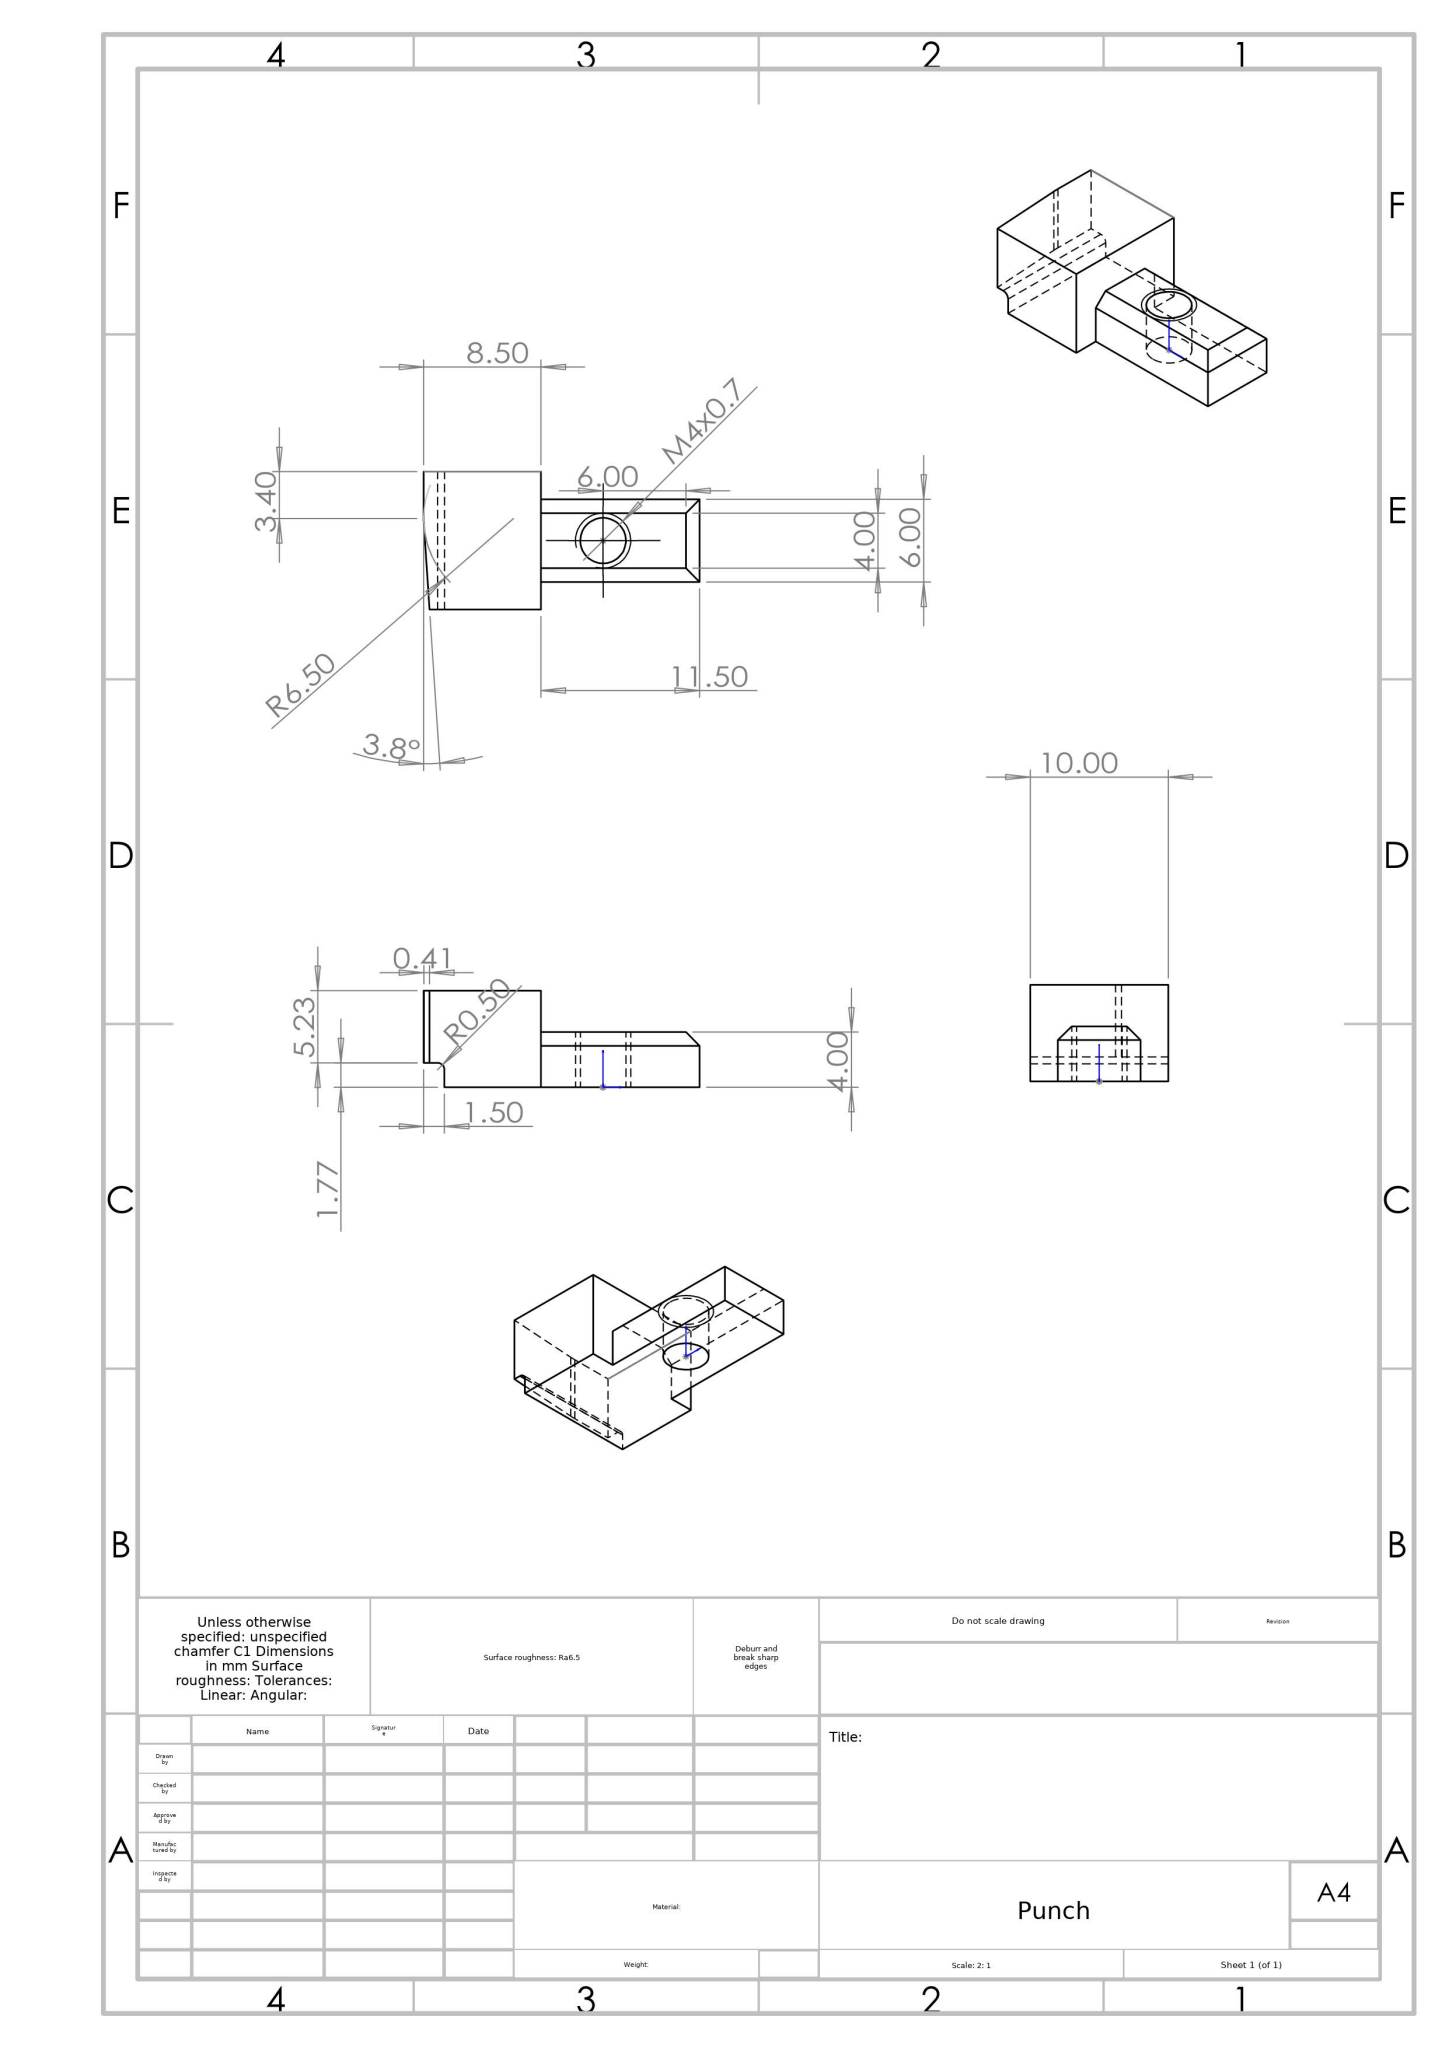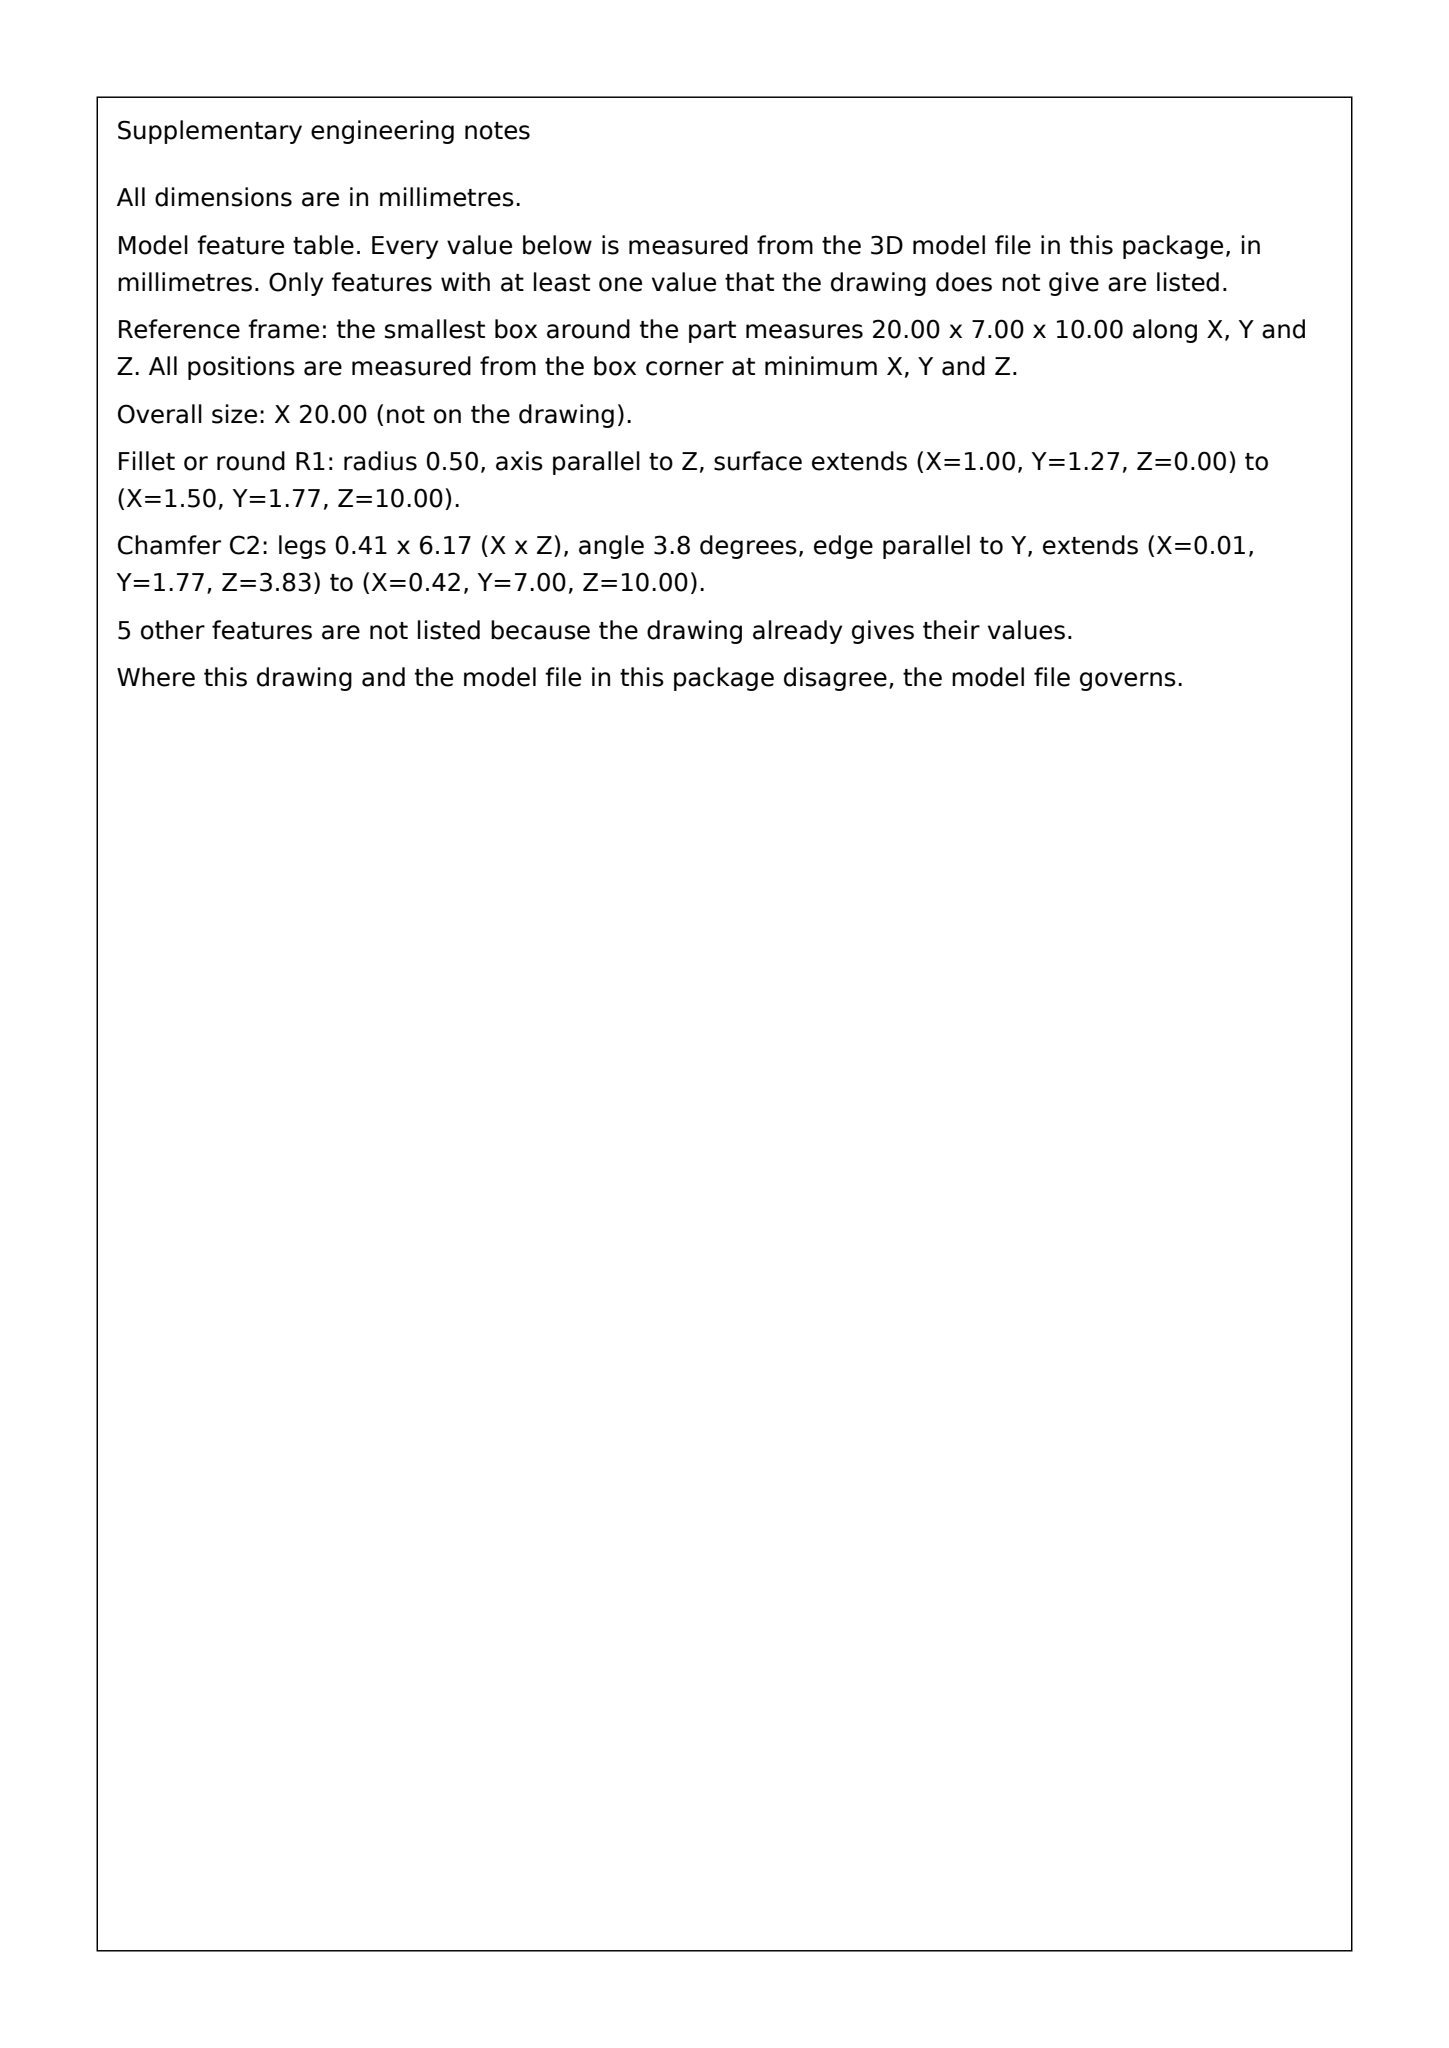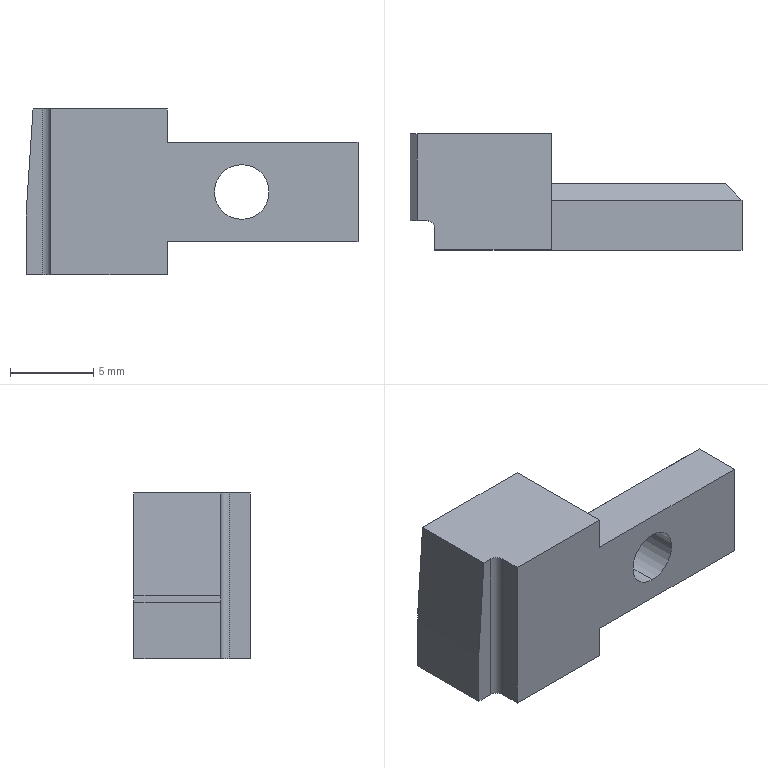Part | SolidWorks | mm | 1 solid | 20 faces | box 20 x 7 x 10 mm | volume 790 mm3 | plane 16 | cylinder 4 | commonest cylinder face diameters 3.3 x2 13 x1 1 x1
STEP:
#1=CARTESIAN_POINT('',(0.,0.,-1.65));
#2=VERTEX_POINT('',#1);
#3=CARTESIAN_POINT('',(0.,0.,1.65));
#4=VERTEX_POINT('',#3);
#5=CARTESIAN_POINT('',(0.,0.,0.));
#6=DIRECTION('',(0.,1.,0.));
#7=DIRECTION('',(0.,0.,1.));
#8=AXIS2_PLACEMENT_3D('',#5,#6,#7);
#9=CIRCLE('',#8,1.65);
#10=EDGE_CURVE('',#2,#4,#9,.T.);
#11=ORIENTED_EDGE('',*,*,#10,.F.);
#12=CARTESIAN_POINT('',(0.,4.,-1.65));
#13=VERTEX_POINT('',#12);
#14=CARTESIAN_POINT('',(0.,4.,-1.65));
#15=DIRECTION('',(0.,1.,0.));
#16=VECTOR('',#15,1000.);
#17=LINE('',#14,#16);
#18=EDGE_CURVE('',#2,#13,#17,.T.);
#19=ORIENTED_EDGE('',*,*,#18,.T.);
#20=CARTESIAN_POINT('',(0.,4.,1.65));
#21=VERTEX_POINT('',#20);
#22=CARTESIAN_POINT('',(0.,4.,0.));
#23=DIRECTION('',(0.,1.,0.));
#24=DIRECTION('',(0.,0.,1.));
#25=AXIS2_PLACEMENT_3D('',#22,#23,#24);
#26=CIRCLE('',#25,1.65);
#27=EDGE_CURVE('',#13,#21,#26,.T.);
#28=ORIENTED_EDGE('',*,*,#27,.T.);
#29=CARTESIAN_POINT('',(0.,4.,1.65));
#30=DIRECTION('',(0.,1.,0.));
#31=VECTOR('',#30,1000.);
#32=LINE('',#29,#31);
#33=EDGE_CURVE('',#4,#21,#32,.T.);
#34=ORIENTED_EDGE('',*,*,#33,.F.);
#35=EDGE_LOOP('',(#11,#19,#28,#34));
#36=FACE_OUTER_BOUND('',#35,.T.);
#37=CARTESIAN_POINT('',(0.,4.,0.));
#38=DIRECTION('',(0.,1.,0.));
#39=DIRECTION('',(0.,0.,1.));
#40=AXIS2_PLACEMENT_3D('',#37,#38,#39);
#41=CYLINDRICAL_SURFACE('',#40,1.65);
#42=ADVANCED_FACE('',(#36),#41,.F.);
#43=CARTESIAN_POINT('',(-13.,7.,-1.6));
#44=VERTEX_POINT('',#43);
#45=CARTESIAN_POINT('',(-12.986,7.,-1.169));
#46=VERTEX_POINT('',#45);
#47=CARTESIAN_POINT('',(-6.5,7.,-1.6));
#48=DIRECTION('',(0.,1.,0.));
#49=DIRECTION('',(0.,0.,1.));
#50=AXIS2_PLACEMENT_3D('',#47,#48,#49);
#51=CIRCLE('',#50,6.5);
#52=EDGE_CURVE('',#44,#46,#51,.T.);
#53=ORIENTED_EDGE('',*,*,#52,.T.);
#54=CARTESIAN_POINT('',(-12.576,7.,5.));
#55=VERTEX_POINT('',#54);
#56=CARTESIAN_POINT('',(-12.852,7.,0.839));
#57=DIRECTION('',(0.06627,0.,0.9978));
#58=VECTOR('',#57,1000.);
#59=LINE('',#56,#58);
#60=EDGE_CURVE('',#46,#55,#59,.T.);
#61=ORIENTED_EDGE('',*,*,#60,.T.);
#62=CARTESIAN_POINT('',(-4.5,7.,5.));
#63=VERTEX_POINT('',#62);
#64=CARTESIAN_POINT('',(-12.78,7.,5.));
#65=DIRECTION('',(1.,0.,0.));
#66=VECTOR('',#65,1000.);
#67=LINE('',#64,#66);
#68=EDGE_CURVE('',#55,#63,#67,.T.);
#69=ORIENTED_EDGE('',*,*,#68,.T.);
#70=CARTESIAN_POINT('',(-4.5,7.,-5.));
#71=VERTEX_POINT('',#70);
#72=CARTESIAN_POINT('',(-4.5,7.,-5.));
#73=DIRECTION('',(0.,0.,-1.));
#74=VECTOR('',#73,1000.);
#75=LINE('',#72,#74);
#76=EDGE_CURVE('',#63,#71,#75,.T.);
#77=ORIENTED_EDGE('',*,*,#76,.T.);
#78=CARTESIAN_POINT('',(-13.,7.,-5.));
#79=VERTEX_POINT('',#78);
#80=CARTESIAN_POINT('',(-12.78,7.,-5.));
#81=DIRECTION('',(1.,0.,0.));
#82=VECTOR('',#81,1000.);
#83=LINE('',#80,#82);
#84=EDGE_CURVE('',#79,#71,#83,.T.);
#85=ORIENTED_EDGE('',*,*,#84,.F.);
#86=CARTESIAN_POINT('',(-13.,7.,-5.));
#87=DIRECTION('',(0.,0.,-1.));
#88=VECTOR('',#87,1000.);
#89=LINE('',#86,#88);
#90=EDGE_CURVE('',#44,#79,#89,.T.);
#91=ORIENTED_EDGE('',*,*,#90,.F.);
#92=EDGE_LOOP('',(#53,#61,#69,#77,#85,#91));
#93=FACE_OUTER_BOUND('',#92,.T.);
#94=CARTESIAN_POINT('',(-12.78,7.,-5.));
#95=DIRECTION('',(0.,-1.,0.));
#96=DIRECTION('',(0.,0.,-1.));
#97=AXIS2_PLACEMENT_3D('',#94,#95,#96);
#98=PLANE('',#97);
#99=ADVANCED_FACE('',(#93),#98,.F.);
#100=CARTESIAN_POINT('',(-12.576,1.77,5.));
#101=VERTEX_POINT('',#100);
#102=CARTESIAN_POINT('',(-12.,1.77,5.));
#103=VERTEX_POINT('',#102);
#104=CARTESIAN_POINT('',(-11.5,1.77,5.));
#105=DIRECTION('',(1.,0.,0.));
#106=VECTOR('',#105,1000.);
#107=LINE('',#104,#106);
#108=EDGE_CURVE('',#101,#103,#107,.T.);
#109=ORIENTED_EDGE('',*,*,#108,.T.);
#110=CARTESIAN_POINT('',(-11.5,1.27,5.));
#111=VERTEX_POINT('',#110);
#112=CARTESIAN_POINT('',(-12.,1.27,5.));
#113=DIRECTION('',(0.,0.,-1.));
#114=DIRECTION('',(-1.,0.,0.));
#115=AXIS2_PLACEMENT_3D('',#112,#113,#114);
#116=CIRCLE('',#115,0.5);
#117=EDGE_CURVE('',#103,#111,#116,.T.);
#118=ORIENTED_EDGE('',*,*,#117,.T.);
#119=CARTESIAN_POINT('',(-11.5,-0.,5.));
#120=VERTEX_POINT('',#119);
#121=CARTESIAN_POINT('',(-11.5,-0.,5.));
#122=DIRECTION('',(0.,-1.,0.));
#123=VECTOR('',#122,1000.);
#124=LINE('',#121,#123);
#125=EDGE_CURVE('',#111,#120,#124,.T.);
#126=ORIENTED_EDGE('',*,*,#125,.T.);
#127=CARTESIAN_POINT('',(-4.5,-0.,5.));
#128=VERTEX_POINT('',#127);
#129=CARTESIAN_POINT('',(-12.78,-0.,5.));
#130=DIRECTION('',(1.,0.,0.));
#131=VECTOR('',#130,1000.);
#132=LINE('',#129,#131);
#133=EDGE_CURVE('',#120,#128,#132,.T.);
#134=ORIENTED_EDGE('',*,*,#133,.T.);
#135=CARTESIAN_POINT('',(-4.5,-0.,5.));
#136=DIRECTION('',(0.,1.,0.));
#137=VECTOR('',#136,1000.);
#138=LINE('',#135,#137);
#139=EDGE_CURVE('',#128,#63,#138,.T.);
#140=ORIENTED_EDGE('',*,*,#139,.T.);
#141=ORIENTED_EDGE('',*,*,#68,.F.);
#142=CARTESIAN_POINT('',(-12.576,-3.,5.));
#143=DIRECTION('',(0.,1.,0.));
#144=VECTOR('',#143,1000.);
#145=LINE('',#142,#144);
#146=EDGE_CURVE('',#101,#55,#145,.T.);
#147=ORIENTED_EDGE('',*,*,#146,.F.);
#148=EDGE_LOOP('',(#109,#118,#126,#134,#140,#141,#147));
#149=FACE_OUTER_BOUND('',#148,.T.);
#150=CARTESIAN_POINT('',(-12.78,-0.,5.));
#151=DIRECTION('',(0.,0.,-1.));
#152=DIRECTION('',(0.,-1.,0.));
#153=AXIS2_PLACEMENT_3D('',#150,#151,#152);
#154=PLANE('',#153);
#155=ADVANCED_FACE('',(#149),#154,.F.);
#156=CARTESIAN_POINT('',(0.,0.,0.));
#157=DIRECTION('',(0.,1.,0.));
#158=DIRECTION('',(0.,0.,1.));
#159=AXIS2_PLACEMENT_3D('',#156,#157,#158);
#160=CIRCLE('',#159,1.65);
#161=EDGE_CURVE('',#4,#2,#160,.T.);
#162=ORIENTED_EDGE('',*,*,#161,.T.);
#163=ORIENTED_EDGE('',*,*,#10,.T.);
#164=EDGE_LOOP('',(#162,#163));
#165=FACE_BOUND('',#164,.T.);
#166=CARTESIAN_POINT('',(-11.5,-0.,-5.));
#167=VERTEX_POINT('',#166);
#168=CARTESIAN_POINT('',(-11.5,-0.,5.));
#169=DIRECTION('',(0.,0.,-1.));
#170=VECTOR('',#169,1000.);
#171=LINE('',#168,#170);
#172=EDGE_CURVE('',#120,#167,#171,.T.);
#173=ORIENTED_EDGE('',*,*,#172,.T.);
#174=CARTESIAN_POINT('',(-4.5,-0.,-5.));
#175=VERTEX_POINT('',#174);
#176=CARTESIAN_POINT('',(-12.78,-0.,-5.));
#177=DIRECTION('',(1.,0.,0.));
#178=VECTOR('',#177,1000.);
#179=LINE('',#176,#178);
#180=EDGE_CURVE('',#167,#175,#179,.T.);
#181=ORIENTED_EDGE('',*,*,#180,.T.);
#182=CARTESIAN_POINT('',(-4.5,0.,-3.));
#183=VERTEX_POINT('',#182);
#184=CARTESIAN_POINT('',(-4.5,-0.,5.));
#185=DIRECTION('',(0.,0.,1.));
#186=VECTOR('',#185,1000.);
#187=LINE('',#184,#186);
#188=EDGE_CURVE('',#175,#183,#187,.T.);
#189=ORIENTED_EDGE('',*,*,#188,.T.);
#190=CARTESIAN_POINT('',(7.,0.,-3.));
#191=VERTEX_POINT('',#190);
#192=CARTESIAN_POINT('',(0.,0.,-3.));
#193=DIRECTION('',(-1.,0.,-0.));
#194=VECTOR('',#193,1000.);
#195=LINE('',#192,#194);
#196=EDGE_CURVE('',#191,#183,#195,.T.);
#197=ORIENTED_EDGE('',*,*,#196,.F.);
#198=CARTESIAN_POINT('',(7.,0.,3.));
#199=VERTEX_POINT('',#198);
#200=CARTESIAN_POINT('',(7.,0.,-3.));
#201=DIRECTION('',(-0.,0.,-1.));
#202=VECTOR('',#201,1000.);
#203=LINE('',#200,#202);
#204=EDGE_CURVE('',#199,#191,#203,.T.);
#205=ORIENTED_EDGE('',*,*,#204,.F.);
#206=CARTESIAN_POINT('',(-4.5,0.,3.));
#207=VERTEX_POINT('',#206);
#208=CARTESIAN_POINT('',(0.,0.,3.));
#209=DIRECTION('',(1.,0.,-0.));
#210=VECTOR('',#209,1000.);
#211=LINE('',#208,#210);
#212=EDGE_CURVE('',#207,#199,#211,.T.);
#213=ORIENTED_EDGE('',*,*,#212,.F.);
#214=CARTESIAN_POINT('',(-4.5,-0.,5.));
#215=DIRECTION('',(0.,0.,1.));
#216=VECTOR('',#215,1000.);
#217=LINE('',#214,#216);
#218=EDGE_CURVE('',#207,#128,#217,.T.);
#219=ORIENTED_EDGE('',*,*,#218,.T.);
#220=ORIENTED_EDGE('',*,*,#133,.F.);
#221=EDGE_LOOP('',(#173,#181,#189,#197,#205,#213,#219,#220));
#222=FACE_OUTER_BOUND('',#221,.T.);
#223=CARTESIAN_POINT('',(0.,0.,0.));
#224=DIRECTION('',(0.,-1.,0.));
#225=DIRECTION('',(0.,0.,-1.));
#226=AXIS2_PLACEMENT_3D('',#223,#224,#225);
#227=PLANE('',#226);
#228=ADVANCED_FACE('',(#165,#222),#227,.T.);
#229=CARTESIAN_POINT('',(-4.5,4.,-2.));
#230=VERTEX_POINT('',#229);
#231=CARTESIAN_POINT('',(-4.5,3.,-3.));
#232=VERTEX_POINT('',#231);
#233=CARTESIAN_POINT('',(-4.5,4.,-2.));
#234=DIRECTION('',(0.,-0.7071,-0.7071));
#235=VECTOR('',#234,1000.);
#236=LINE('',#233,#235);
#237=EDGE_CURVE('',#230,#232,#236,.T.);
#238=ORIENTED_EDGE('',*,*,#237,.T.);
#239=CARTESIAN_POINT('',(-4.5,4.,-3.));
#240=DIRECTION('',(0.,-1.,0.));
#241=VECTOR('',#240,1000.);
#242=LINE('',#239,#241);
#243=EDGE_CURVE('',#232,#183,#242,.T.);
#244=ORIENTED_EDGE('',*,*,#243,.T.);
#245=ORIENTED_EDGE('',*,*,#188,.F.);
#246=CARTESIAN_POINT('',(-4.5,-0.,-5.));
#247=DIRECTION('',(0.,-1.,0.));
#248=VECTOR('',#247,1000.);
#249=LINE('',#246,#248);
#250=EDGE_CURVE('',#71,#175,#249,.T.);
#251=ORIENTED_EDGE('',*,*,#250,.F.);
#252=ORIENTED_EDGE('',*,*,#76,.F.);
#253=ORIENTED_EDGE('',*,*,#139,.F.);
#254=ORIENTED_EDGE('',*,*,#218,.F.);
#255=CARTESIAN_POINT('',(-4.5,3.,3.));
#256=VERTEX_POINT('',#255);
#257=CARTESIAN_POINT('',(-4.5,4.,3.));
#258=DIRECTION('',(0.,-1.,0.));
#259=VECTOR('',#258,1000.);
#260=LINE('',#257,#259);
#261=EDGE_CURVE('',#256,#207,#260,.T.);
#262=ORIENTED_EDGE('',*,*,#261,.F.);
#263=CARTESIAN_POINT('',(-4.5,4.,2.));
#264=VERTEX_POINT('',#263);
#265=CARTESIAN_POINT('',(-4.5,4.,2.));
#266=DIRECTION('',(0.,0.7071,-0.7071));
#267=VECTOR('',#266,1000.);
#268=LINE('',#265,#267);
#269=EDGE_CURVE('',#256,#264,#268,.T.);
#270=ORIENTED_EDGE('',*,*,#269,.T.);
#271=CARTESIAN_POINT('',(-4.5,4.,3.));
#272=DIRECTION('',(0.,0.,1.));
#273=VECTOR('',#272,1000.);
#274=LINE('',#271,#273);
#275=EDGE_CURVE('',#230,#264,#274,.T.);
#276=ORIENTED_EDGE('',*,*,#275,.F.);
#277=EDGE_LOOP('',(#238,#244,#245,#251,#252,#253,#254,#262,#270,#276));
#278=FACE_OUTER_BOUND('',#277,.T.);
#279=CARTESIAN_POINT('',(-4.5,0.,0.));
#280=DIRECTION('',(1.,0.,0.));
#281=DIRECTION('',(0.,1.,0.));
#282=AXIS2_PLACEMENT_3D('',#279,#280,#281);
#283=PLANE('',#282);
#284=ADVANCED_FACE('',(#278),#283,.T.);
#285=CARTESIAN_POINT('',(-13.,1.77,-5.));
#286=VERTEX_POINT('',#285);
#287=CARTESIAN_POINT('',(-13.,-0.,-5.));
#288=DIRECTION('',(0.,-1.,0.));
#289=VECTOR('',#288,1000.);
#290=LINE('',#287,#289);
#291=EDGE_CURVE('',#79,#286,#290,.T.);
#292=ORIENTED_EDGE('',*,*,#291,.T.);
#293=CARTESIAN_POINT('',(-13.,1.77,-1.6));
#294=VERTEX_POINT('',#293);
#295=CARTESIAN_POINT('',(-13.,1.77,5.));
#296=DIRECTION('',(0.,0.,-1.));
#297=VECTOR('',#296,1000.);
#298=LINE('',#295,#297);
#299=EDGE_CURVE('',#294,#286,#298,.T.);
#300=ORIENTED_EDGE('',*,*,#299,.F.);
#301=CARTESIAN_POINT('',(-13.,-3.,-1.6));
#302=DIRECTION('',(0.,1.,0.));
#303=VECTOR('',#302,1000.);
#304=LINE('',#301,#303);
#305=EDGE_CURVE('',#294,#44,#304,.T.);
#306=ORIENTED_EDGE('',*,*,#305,.T.);
#307=ORIENTED_EDGE('',*,*,#90,.T.);
#308=EDGE_LOOP('',(#292,#300,#306,#307));
#309=FACE_OUTER_BOUND('',#308,.T.);
#310=CARTESIAN_POINT('',(-13.,0.,0.));
#311=DIRECTION('',(1.,0.,0.));
#312=DIRECTION('',(0.,1.,0.));
#313=AXIS2_PLACEMENT_3D('',#310,#311,#312);
#314=PLANE('',#313);
#315=ADVANCED_FACE('',(#309),#314,.F.);
#316=ORIENTED_EDGE('',*,*,#180,.F.);
#317=CARTESIAN_POINT('',(-11.5,1.27,-5.));
#318=VERTEX_POINT('',#317);
#319=CARTESIAN_POINT('',(-11.5,-0.,-5.));
#320=DIRECTION('',(0.,-1.,0.));
#321=VECTOR('',#320,1000.);
#322=LINE('',#319,#321);
#323=EDGE_CURVE('',#318,#167,#322,.T.);
#324=ORIENTED_EDGE('',*,*,#323,.F.);
#325=CARTESIAN_POINT('',(-12.,1.77,-5.));
#326=VERTEX_POINT('',#325);
#327=CARTESIAN_POINT('',(-12.,1.27,-5.));
#328=DIRECTION('',(0.,0.,1.));
#329=DIRECTION('',(1.,0.,0.));
#330=AXIS2_PLACEMENT_3D('',#327,#328,#329);
#331=CIRCLE('',#330,0.5);
#332=EDGE_CURVE('',#318,#326,#331,.T.);
#333=ORIENTED_EDGE('',*,*,#332,.T.);
#334=CARTESIAN_POINT('',(-11.5,1.77,-5.));
#335=DIRECTION('',(1.,0.,0.));
#336=VECTOR('',#335,1000.);
#337=LINE('',#334,#336);
#338=EDGE_CURVE('',#286,#326,#337,.T.);
#339=ORIENTED_EDGE('',*,*,#338,.F.);
#340=ORIENTED_EDGE('',*,*,#291,.F.);
#341=ORIENTED_EDGE('',*,*,#84,.T.);
#342=ORIENTED_EDGE('',*,*,#250,.T.);
#343=EDGE_LOOP('',(#316,#324,#333,#339,#340,#341,#342));
#344=FACE_OUTER_BOUND('',#343,.T.);
#345=CARTESIAN_POINT('',(-12.78,-0.,-5.));
#346=DIRECTION('',(0.,0.,1.));
#347=DIRECTION('',(1.,0.,0.));
#348=AXIS2_PLACEMENT_3D('',#345,#346,#347);
#349=PLANE('',#348);
#350=ADVANCED_FACE('',(#344),#349,.F.);
#351=CARTESIAN_POINT('',(6.,4.,-2.));
#352=VERTEX_POINT('',#351);
#353=CARTESIAN_POINT('',(7.,3.,-3.));
#354=VERTEX_POINT('',#353);
#355=CARTESIAN_POINT('',(5.333,4.667,-1.333));
#356=DIRECTION('',(0.5774,-0.5774,-0.5774));
#357=VECTOR('',#356,1000.);
#358=LINE('',#355,#357);
#359=EDGE_CURVE('',#352,#354,#358,.T.);
#360=ORIENTED_EDGE('',*,*,#359,.T.);
#361=CARTESIAN_POINT('',(0.,3.,-3.));
#362=DIRECTION('',(1.,0.,0.));
#363=VECTOR('',#362,1000.);
#364=LINE('',#361,#363);
#365=EDGE_CURVE('',#232,#354,#364,.T.);
#366=ORIENTED_EDGE('',*,*,#365,.F.);
#367=ORIENTED_EDGE('',*,*,#237,.F.);
#368=CARTESIAN_POINT('',(0.,4.,-2.));
#369=DIRECTION('',(-1.,0.,-0.));
#370=VECTOR('',#369,1000.);
#371=LINE('',#368,#370);
#372=EDGE_CURVE('',#352,#230,#371,.T.);
#373=ORIENTED_EDGE('',*,*,#372,.F.);
#374=EDGE_LOOP('',(#360,#366,#367,#373));
#375=FACE_OUTER_BOUND('',#374,.T.);
#376=CARTESIAN_POINT('',(0.,4.,-2.));
#377=DIRECTION('',(-0.,-0.7071,0.7071));
#378=DIRECTION('',(-1.,0.,0.));
#379=AXIS2_PLACEMENT_3D('',#376,#377,#378);
#380=PLANE('',#379);
#381=ADVANCED_FACE('',(#375),#380,.F.);
#382=CARTESIAN_POINT('',(6.,4.,2.));
#383=VERTEX_POINT('',#382);
#384=CARTESIAN_POINT('',(7.,3.,3.));
#385=VERTEX_POINT('',#384);
#386=CARTESIAN_POINT('',(4.,6.,0.));
#387=DIRECTION('',(0.5774,-0.5774,0.5774));
#388=VECTOR('',#387,1000.);
#389=LINE('',#386,#388);
#390=EDGE_CURVE('',#383,#385,#389,.T.);
#391=ORIENTED_EDGE('',*,*,#390,.T.);
#392=CARTESIAN_POINT('',(7.,3.,-3.));
#393=DIRECTION('',(0.,0.,1.));
#394=VECTOR('',#393,1000.);
#395=LINE('',#392,#394);
#396=EDGE_CURVE('',#354,#385,#395,.T.);
#397=ORIENTED_EDGE('',*,*,#396,.F.);
#398=ORIENTED_EDGE('',*,*,#359,.F.);
#399=CARTESIAN_POINT('',(6.,4.,-0.));
#400=DIRECTION('',(-0.,0.,-1.));
#401=VECTOR('',#400,1000.);
#402=LINE('',#399,#401);
#403=EDGE_CURVE('',#383,#352,#402,.T.);
#404=ORIENTED_EDGE('',*,*,#403,.F.);
#405=EDGE_LOOP('',(#391,#397,#398,#404));
#406=FACE_OUTER_BOUND('',#405,.T.);
#407=CARTESIAN_POINT('',(6.,4.,-0.));
#408=DIRECTION('',(-0.7071,-0.7071,0.));
#409=DIRECTION('',(-0.7071,0.7071,0.));
#410=AXIS2_PLACEMENT_3D('',#407,#408,#409);
#411=PLANE('',#410);
#412=ADVANCED_FACE('',(#406),#411,.F.);
#413=ORIENTED_EDGE('',*,*,#269,.F.);
#414=CARTESIAN_POINT('',(0.,3.,3.));
#415=DIRECTION('',(-1.,0.,0.));
#416=VECTOR('',#415,1000.);
#417=LINE('',#414,#416);
#418=EDGE_CURVE('',#385,#256,#417,.T.);
#419=ORIENTED_EDGE('',*,*,#418,.F.);
#420=ORIENTED_EDGE('',*,*,#390,.F.);
#421=CARTESIAN_POINT('',(0.,4.,2.));
#422=DIRECTION('',(1.,0.,-0.));
#423=VECTOR('',#422,1000.);
#424=LINE('',#421,#423);
#425=EDGE_CURVE('',#264,#383,#424,.T.);
#426=ORIENTED_EDGE('',*,*,#425,.F.);
#427=EDGE_LOOP('',(#413,#419,#420,#426));
#428=FACE_OUTER_BOUND('',#427,.T.);
#429=CARTESIAN_POINT('',(0.,4.,2.));
#430=DIRECTION('',(-0.,-0.7071,-0.7071));
#431=DIRECTION('',(0.,-0.7071,0.7071));
#432=AXIS2_PLACEMENT_3D('',#429,#430,#431);
#433=PLANE('',#432);
#434=ADVANCED_FACE('',(#428),#433,.F.);
#435=CARTESIAN_POINT('',(0.,4.,0.));
#436=DIRECTION('',(0.,1.,0.));
#437=DIRECTION('',(0.,0.,1.));
#438=AXIS2_PLACEMENT_3D('',#435,#436,#437);
#439=CIRCLE('',#438,1.65);
#440=EDGE_CURVE('',#21,#13,#439,.T.);
#441=ORIENTED_EDGE('',*,*,#440,.F.);
#442=ORIENTED_EDGE('',*,*,#27,.F.);
#443=EDGE_LOOP('',(#441,#442));
#444=FACE_BOUND('',#443,.T.);
#445=ORIENTED_EDGE('',*,*,#403,.T.);
#446=ORIENTED_EDGE('',*,*,#372,.T.);
#447=ORIENTED_EDGE('',*,*,#275,.T.);
#448=ORIENTED_EDGE('',*,*,#425,.T.);
#449=EDGE_LOOP('',(#445,#446,#447,#448));
#450=FACE_OUTER_BOUND('',#449,.T.);
#451=CARTESIAN_POINT('',(0.,4.,0.));
#452=DIRECTION('',(0.,-1.,0.));
#453=DIRECTION('',(0.,0.,-1.));
#454=AXIS2_PLACEMENT_3D('',#451,#452,#453);
#455=PLANE('',#454);
#456=ADVANCED_FACE('',(#444,#450),#455,.F.);
#457=ORIENTED_EDGE('',*,*,#243,.F.);
#458=ORIENTED_EDGE('',*,*,#365,.T.);
#459=CARTESIAN_POINT('',(7.,4.,-3.));
#460=DIRECTION('',(0.,-1.,0.));
#461=VECTOR('',#460,1000.);
#462=LINE('',#459,#461);
#463=EDGE_CURVE('',#354,#191,#462,.T.);
#464=ORIENTED_EDGE('',*,*,#463,.T.);
#465=ORIENTED_EDGE('',*,*,#196,.T.);
#466=EDGE_LOOP('',(#457,#458,#464,#465));
#467=FACE_OUTER_BOUND('',#466,.T.);
#468=CARTESIAN_POINT('',(0.,4.,-3.));
#469=DIRECTION('',(-0.,0.,1.));
#470=DIRECTION('',(1.,0.,0.));
#471=AXIS2_PLACEMENT_3D('',#468,#469,#470);
#472=PLANE('',#471);
#473=ADVANCED_FACE('',(#467),#472,.F.);
#474=ORIENTED_EDGE('',*,*,#463,.F.);
#475=ORIENTED_EDGE('',*,*,#396,.T.);
#476=CARTESIAN_POINT('',(7.,4.,3.));
#477=DIRECTION('',(0.,-1.,0.));
#478=VECTOR('',#477,1000.);
#479=LINE('',#476,#478);
#480=EDGE_CURVE('',#385,#199,#479,.T.);
#481=ORIENTED_EDGE('',*,*,#480,.T.);
#482=ORIENTED_EDGE('',*,*,#204,.T.);
#483=EDGE_LOOP('',(#474,#475,#481,#482));
#484=FACE_OUTER_BOUND('',#483,.T.);
#485=CARTESIAN_POINT('',(7.,4.,-3.));
#486=DIRECTION('',(-1.,0.,0.));
#487=DIRECTION('',(0.,1.,0.));
#488=AXIS2_PLACEMENT_3D('',#485,#486,#487);
#489=PLANE('',#488);
#490=ADVANCED_FACE('',(#484),#489,.F.);
#491=ORIENTED_EDGE('',*,*,#480,.F.);
#492=ORIENTED_EDGE('',*,*,#418,.T.);
#493=ORIENTED_EDGE('',*,*,#261,.T.);
#494=ORIENTED_EDGE('',*,*,#212,.T.);
#495=EDGE_LOOP('',(#491,#492,#493,#494));
#496=FACE_OUTER_BOUND('',#495,.T.);
#497=CARTESIAN_POINT('',(0.,4.,3.));
#498=DIRECTION('',(-0.,0.,-1.));
#499=DIRECTION('',(-1.,0.,0.));
#500=AXIS2_PLACEMENT_3D('',#497,#498,#499);
#501=PLANE('',#500);
#502=ADVANCED_FACE('',(#496),#501,.F.);
#503=CARTESIAN_POINT('',(-12.986,1.77,-1.169));
#504=VERTEX_POINT('',#503);
#505=CARTESIAN_POINT('',(-6.5,1.77,-1.6));
#506=DIRECTION('',(0.,-1.,0.));
#507=DIRECTION('',(0.,0.,1.));
#508=AXIS2_PLACEMENT_3D('',#505,#506,#507);
#509=CIRCLE('',#508,6.5);
#510=EDGE_CURVE('',#504,#294,#509,.T.);
#511=ORIENTED_EDGE('',*,*,#510,.F.);
#512=CARTESIAN_POINT('',(-12.986,-3.,-1.169));
#513=DIRECTION('',(0.,1.,0.));
#514=VECTOR('',#513,1000.);
#515=LINE('',#512,#514);
#516=EDGE_CURVE('',#504,#46,#515,.T.);
#517=ORIENTED_EDGE('',*,*,#516,.T.);
#518=ORIENTED_EDGE('',*,*,#52,.F.);
#519=ORIENTED_EDGE('',*,*,#305,.F.);
#520=EDGE_LOOP('',(#511,#517,#518,#519));
#521=FACE_OUTER_BOUND('',#520,.T.);
#522=CARTESIAN_POINT('',(-6.5,-3.,-1.6));
#523=DIRECTION('',(0.,1.,0.));
#524=DIRECTION('',(0.,0.,1.));
#525=AXIS2_PLACEMENT_3D('',#522,#523,#524);
#526=CYLINDRICAL_SURFACE('',#525,6.5);
#527=ADVANCED_FACE('',(#521),#526,.T.);
#528=CARTESIAN_POINT('',(-12.852,1.77,0.839));
#529=DIRECTION('',(-0.06627,0.,-0.9978));
#530=VECTOR('',#529,1000.);
#531=LINE('',#528,#530);
#532=EDGE_CURVE('',#101,#504,#531,.T.);
#533=ORIENTED_EDGE('',*,*,#532,.F.);
#534=ORIENTED_EDGE('',*,*,#146,.T.);
#535=ORIENTED_EDGE('',*,*,#60,.F.);
#536=ORIENTED_EDGE('',*,*,#516,.F.);
#537=EDGE_LOOP('',(#533,#534,#535,#536));
#538=FACE_OUTER_BOUND('',#537,.T.);
#539=CARTESIAN_POINT('',(-12.852,-3.,0.839));
#540=DIRECTION('',(-0.9978,0.,0.06627));
#541=DIRECTION('',(0.06627,0.,0.9978));
#542=AXIS2_PLACEMENT_3D('',#539,#540,#541);
#543=PLANE('',#542);
#544=ADVANCED_FACE('',(#538),#543,.T.);
#545=ORIENTED_EDGE('',*,*,#125,.F.);
#546=CARTESIAN_POINT('',(-11.5,1.27,-5.));
#547=DIRECTION('',(0.,0.,-1.));
#548=VECTOR('',#547,1000.);
#549=LINE('',#546,#548);
#550=EDGE_CURVE('',#111,#318,#549,.T.);
#551=ORIENTED_EDGE('',*,*,#550,.T.);
#552=ORIENTED_EDGE('',*,*,#323,.T.);
#553=ORIENTED_EDGE('',*,*,#172,.F.);
#554=EDGE_LOOP('',(#545,#551,#552,#553));
#555=FACE_OUTER_BOUND('',#554,.T.);
#556=CARTESIAN_POINT('',(-11.5,-0.,5.));
#557=DIRECTION('',(1.,0.,0.));
#558=DIRECTION('',(0.,0.,-1.));
#559=AXIS2_PLACEMENT_3D('',#556,#557,#558);
#560=PLANE('',#559);
#561=ADVANCED_FACE('',(#555),#560,.F.);
#562=ORIENTED_EDGE('',*,*,#338,.T.);
#563=CARTESIAN_POINT('',(-12.,1.77,5.));
#564=DIRECTION('',(0.,0.,1.));
#565=VECTOR('',#564,1000.);
#566=LINE('',#563,#565);
#567=EDGE_CURVE('',#326,#103,#566,.T.);
#568=ORIENTED_EDGE('',*,*,#567,.T.);
#569=ORIENTED_EDGE('',*,*,#108,.F.);
#570=ORIENTED_EDGE('',*,*,#532,.T.);
#571=ORIENTED_EDGE('',*,*,#510,.T.);
#572=ORIENTED_EDGE('',*,*,#299,.T.);
#573=EDGE_LOOP('',(#562,#568,#569,#570,#571,#572));
#574=FACE_OUTER_BOUND('',#573,.T.);
#575=CARTESIAN_POINT('',(-11.5,1.77,5.));
#576=DIRECTION('',(0.,1.,0.));
#577=DIRECTION('',(0.,0.,1.));
#578=AXIS2_PLACEMENT_3D('',#575,#576,#577);
#579=PLANE('',#578);
#580=ADVANCED_FACE('',(#574),#579,.F.);
#581=ORIENTED_EDGE('',*,*,#117,.F.);
#582=ORIENTED_EDGE('',*,*,#567,.F.);
#583=ORIENTED_EDGE('',*,*,#332,.F.);
#584=ORIENTED_EDGE('',*,*,#550,.F.);
#585=EDGE_LOOP('',(#581,#582,#583,#584));
#586=FACE_OUTER_BOUND('',#585,.T.);
#587=CARTESIAN_POINT('',(-12.,1.27,5.));
#588=DIRECTION('',(0.,0.,1.));
#589=DIRECTION('',(1.,0.,0.));
#590=AXIS2_PLACEMENT_3D('',#587,#588,#589);
#591=CYLINDRICAL_SURFACE('',#590,0.5);
#592=ADVANCED_FACE('',(#586),#591,.F.);
#593=ORIENTED_EDGE('',*,*,#18,.F.);
#594=ORIENTED_EDGE('',*,*,#161,.F.);
#595=ORIENTED_EDGE('',*,*,#33,.T.);
#596=ORIENTED_EDGE('',*,*,#440,.T.);
#597=EDGE_LOOP('',(#593,#594,#595,#596));
#598=FACE_OUTER_BOUND('',#597,.T.);
#599=CARTESIAN_POINT('',(0.,4.,0.));
#600=DIRECTION('',(0.,1.,0.));
#601=DIRECTION('',(0.,0.,1.));
#602=AXIS2_PLACEMENT_3D('',#599,#600,#601);
#603=CYLINDRICAL_SURFACE('',#602,1.65);
#604=ADVANCED_FACE('',(#598),#603,.F.);
#605=CLOSED_SHELL('',(#42,#99,#155,#228,#284,#315,#350,#381,#412,#434,#456,#473,#490,#502,#527,#544,#561,#580,#592,#604));
#606=MANIFOLD_SOLID_BREP('',#605);
#607=CARTESIAN_POINT('',(0.,0.,0.));
#608=DIRECTION('',(0.,0.,1.));
#609=DIRECTION('',(1.,0.,0.));
#610=AXIS2_PLACEMENT_3D('',#607,#608,#609);
#611=(LENGTH_UNIT()NAMED_UNIT(*)SI_UNIT(.MILLI.,.METRE.));
#612=UNCERTAINTY_MEASURE_WITH_UNIT(LENGTH_MEASURE(0.00001),#611,'','');
#613=(NAMED_UNIT(*)PLANE_ANGLE_UNIT()SI_UNIT($,.RADIAN.));
#614=(NAMED_UNIT(*)SI_UNIT($,.STERADIAN.)SOLID_ANGLE_UNIT());
#615=(GEOMETRIC_REPRESENTATION_CONTEXT(3)GLOBAL_UNCERTAINTY_ASSIGNED_CONTEXT((#612))GLOBAL_UNIT_ASSIGNED_CONTEXT((#611,#613,#614))REPRESENTATION_CONTEXT('',''));
#616=ADVANCED_BREP_SHAPE_REPRESENTATION('',(#606,#610),#615);